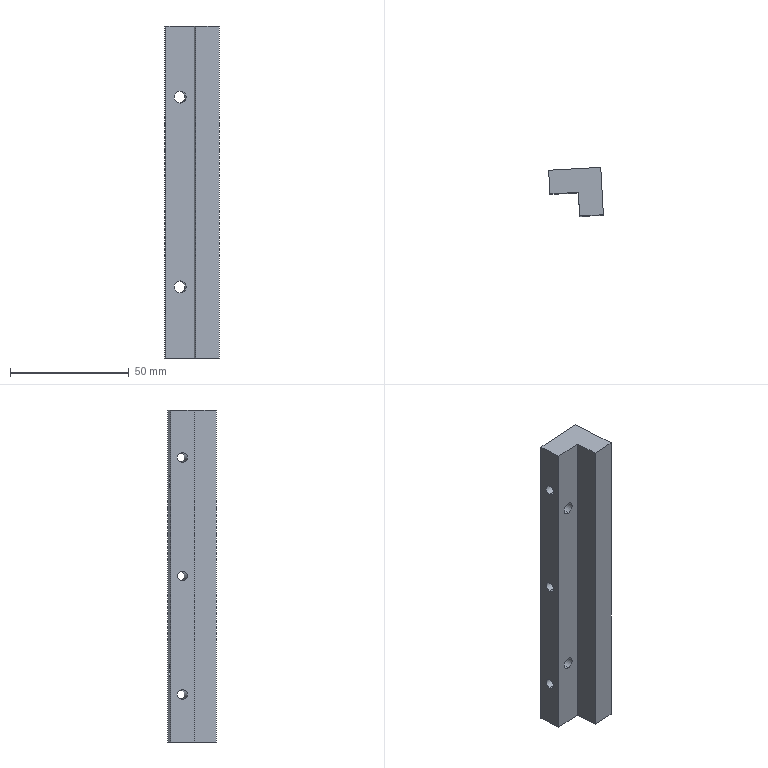Component | SolidWorks | BearingPressPartH-1 | 1 solid | 18 faces | box 23.06 x 20.52 x 140 mm | volume 43493 mm3 | cylinder 10 | plane 8 | commonest cylinder face diameters 4.2 x6 5 x4
build123d program:
from build123d import *

# Parameters (mm, degrees)
BOSS_EXTRUDE1_DEPTH   = 140
M5_TAPPED_HOLE1_D     = 4.2
M6_TAPPED_HOLE1_D     = 5
M6_TAPPED_HOLE1_DEPTH = 36.5
M6_TAPPED_HOLE1_TIP   = 1.502


with BuildPart() as part:
    # Sketch1 → Boss-Extrude1 (new body)
    with BuildSketch(Plane.XY):
        Polygon((0, 0), (10, 0), (10, 20), (-12, 20), (-12, 10), (0, 10), align=None)
    extrude(amount=BOSS_EXTRUDE1_DEPTH)

    # M5 Tapped Hole1 (through all)
    with Locations(Plane(origin=(10, 0, 0), x_dir=(0, 0, -1), z_dir=(1, 0, 0))):
        with Locations((-120, 15), (-70, 15), (-20, 15)):
            Hole(M5_TAPPED_HOLE1_D / 2)

    # M6 Tapped Hole1
    with Locations(Plane(origin=(0, 20, 0), x_dir=(1, 0, 0), z_dir=(0, 1, 0))):
        with Locations((-6, -110), (-6, -30)):
            Hole(M6_TAPPED_HOLE1_D / 2, depth=M6_TAPPED_HOLE1_DEPTH)
            with Locations((0, 0, -(M6_TAPPED_HOLE1_DEPTH + M6_TAPPED_HOLE1_TIP / 2))):  # 118° drill point
                Cone(0, M6_TAPPED_HOLE1_D / 2, M6_TAPPED_HOLE1_TIP, mode=Mode.SUBTRACT)


solid = part.part

# Placed as in the assembly
solid = solid.moved(Location((403.598, 155.593, -283.818), (0, 0, 3.137)))
STEP:
#1=COLOUR_RGB('',0.7922,0.8196,0.9333);
#2=FILL_AREA_STYLE_COLOUR('',#1);
#3=FILL_AREA_STYLE('',(#2));
#4=SURFACE_STYLE_FILL_AREA(#3);
#5=SURFACE_SIDE_STYLE('',(#4));
#6=SURFACE_STYLE_USAGE(.BOTH.,#5);
#7=PRESENTATION_STYLE_ASSIGNMENT((#6));
#8=CARTESIAN_POINT('',(15.632,6.506,-6.942));
#9=VERTEX_POINT('',#8);
#10=CARTESIAN_POINT('',(15.632,6.506,-6.745));
#11=VERTEX_POINT('',#10);
#12=CARTESIAN_POINT('',(15.632,6.506,-6.843));
#13=DIRECTION('',(-0.05472,0.9985,-0.));
#14=DIRECTION('',(0.,0.,1.));
#15=AXIS2_PLACEMENT_3D('',#12,#13,#14);
#16=CIRCLE('',#15,0.09843);
#17=EDGE_CURVE('',#9,#11,#16,.T.);
#18=ORIENTED_EDGE('',*,*,#17,.F.);
#19=CARTESIAN_POINT('',(15.611,6.899,-6.942));
#20=VERTEX_POINT('',#19);
#21=CARTESIAN_POINT('',(15.611,6.899,-6.942));
#22=DIRECTION('',(-0.05472,0.9985,-0.));
#23=VECTOR('',#22,39.37);
#24=LINE('',#21,#23);
#25=EDGE_CURVE('',#9,#20,#24,.T.);
#26=ORIENTED_EDGE('',*,*,#25,.T.);
#27=CARTESIAN_POINT('',(15.611,6.899,-6.745));
#28=VERTEX_POINT('',#27);
#29=CARTESIAN_POINT('',(15.611,6.899,-6.843));
#30=DIRECTION('',(-0.05472,0.9985,-0.));
#31=DIRECTION('',(0.,0.,1.));
#32=AXIS2_PLACEMENT_3D('',#29,#30,#31);
#33=CIRCLE('',#32,0.09843);
#34=EDGE_CURVE('',#20,#28,#33,.T.);
#35=ORIENTED_EDGE('',*,*,#34,.T.);
#36=CARTESIAN_POINT('',(15.611,6.899,-6.745));
#37=DIRECTION('',(-0.05472,0.9985,-0.));
#38=VECTOR('',#37,39.37);
#39=LINE('',#36,#38);
#40=EDGE_CURVE('',#11,#28,#39,.T.);
#41=ORIENTED_EDGE('',*,*,#40,.F.);
#42=EDGE_LOOP('',(#18,#26,#35,#41));
#43=FACE_OUTER_BOUND('',#42,.T.);
#44=CARTESIAN_POINT('',(15.611,6.899,-6.843));
#45=DIRECTION('',(-0.05472,0.9985,-0.));
#46=DIRECTION('',(0.,0.,1.));
#47=AXIS2_PLACEMENT_3D('',#44,#45,#46);
#48=CYLINDRICAL_SURFACE('',#47,0.09843);
#49=ADVANCED_FACE('',(#43),#48,.F.);
#50=CARTESIAN_POINT('',(15.632,6.506,-10.091));
#51=VERTEX_POINT('',#50);
#52=CARTESIAN_POINT('',(15.632,6.506,-9.894));
#53=VERTEX_POINT('',#52);
#54=CARTESIAN_POINT('',(15.632,6.506,-9.993));
#55=DIRECTION('',(-0.05472,0.9985,-0.));
#56=DIRECTION('',(0.,0.,1.));
#57=AXIS2_PLACEMENT_3D('',#54,#55,#56);
#58=CIRCLE('',#57,0.09843);
#59=EDGE_CURVE('',#51,#53,#58,.T.);
#60=ORIENTED_EDGE('',*,*,#59,.F.);
#61=CARTESIAN_POINT('',(15.611,6.899,-10.091));
#62=VERTEX_POINT('',#61);
#63=CARTESIAN_POINT('',(15.611,6.899,-10.091));
#64=DIRECTION('',(-0.05472,0.9985,-0.));
#65=VECTOR('',#64,39.37);
#66=LINE('',#63,#65);
#67=EDGE_CURVE('',#51,#62,#66,.T.);
#68=ORIENTED_EDGE('',*,*,#67,.T.);
#69=CARTESIAN_POINT('',(15.611,6.899,-9.894));
#70=VERTEX_POINT('',#69);
#71=CARTESIAN_POINT('',(15.611,6.899,-9.993));
#72=DIRECTION('',(-0.05472,0.9985,-0.));
#73=DIRECTION('',(0.,0.,1.));
#74=AXIS2_PLACEMENT_3D('',#71,#72,#73);
#75=CIRCLE('',#74,0.09843);
#76=EDGE_CURVE('',#62,#70,#75,.T.);
#77=ORIENTED_EDGE('',*,*,#76,.T.);
#78=CARTESIAN_POINT('',(15.611,6.899,-9.894));
#79=DIRECTION('',(-0.05472,0.9985,-0.));
#80=VECTOR('',#79,39.37);
#81=LINE('',#78,#80);
#82=EDGE_CURVE('',#53,#70,#81,.T.);
#83=ORIENTED_EDGE('',*,*,#82,.F.);
#84=EDGE_LOOP('',(#60,#68,#77,#83));
#85=FACE_OUTER_BOUND('',#84,.T.);
#86=CARTESIAN_POINT('',(15.611,6.899,-9.993));
#87=DIRECTION('',(-0.05472,0.9985,-0.));
#88=DIRECTION('',(0.,0.,1.));
#89=AXIS2_PLACEMENT_3D('',#86,#87,#88);
#90=CYLINDRICAL_SURFACE('',#89,0.09843);
#91=ADVANCED_FACE('',(#85),#90,.F.);
#92=CARTESIAN_POINT('',(15.386,6.69,-6.367));
#93=VERTEX_POINT('',#92);
#94=CARTESIAN_POINT('',(15.386,6.69,-6.532));
#95=VERTEX_POINT('',#94);
#96=CARTESIAN_POINT('',(15.386,6.69,-6.45));
#97=DIRECTION('',(0.9985,0.05472,-0.));
#98=DIRECTION('',(-0.05472,0.9985,0.));
#99=AXIS2_PLACEMENT_3D('',#96,#97,#98);
#100=CIRCLE('',#99,0.08268);
#101=EDGE_CURVE('',#93,#95,#100,.T.);
#102=ORIENTED_EDGE('',*,*,#101,.F.);
#103=CARTESIAN_POINT('',(16.251,6.737,-6.367));
#104=VERTEX_POINT('',#103);
#105=CARTESIAN_POINT('',(16.251,6.737,-6.367));
#106=DIRECTION('',(0.9985,0.05472,-0.));
#107=VECTOR('',#106,39.37);
#108=LINE('',#105,#107);
#109=EDGE_CURVE('',#93,#104,#108,.T.);
#110=ORIENTED_EDGE('',*,*,#109,.T.);
#111=CARTESIAN_POINT('',(16.251,6.737,-6.532));
#112=VERTEX_POINT('',#111);
#113=CARTESIAN_POINT('',(16.251,6.737,-6.45));
#114=DIRECTION('',(0.9985,0.05472,-0.));
#115=DIRECTION('',(0.,0.,-1.));
#116=AXIS2_PLACEMENT_3D('',#113,#114,#115);
#117=CIRCLE('',#116,0.08268);
#118=EDGE_CURVE('',#104,#112,#117,.T.);
#119=ORIENTED_EDGE('',*,*,#118,.T.);
#120=CARTESIAN_POINT('',(16.251,6.737,-6.532));
#121=DIRECTION('',(0.9985,0.05472,-0.));
#122=VECTOR('',#121,39.37);
#123=LINE('',#120,#122);
#124=EDGE_CURVE('',#95,#112,#123,.T.);
#125=ORIENTED_EDGE('',*,*,#124,.F.);
#126=EDGE_LOOP('',(#102,#110,#119,#125));
#127=FACE_OUTER_BOUND('',#126,.T.);
#128=CARTESIAN_POINT('',(16.251,6.737,-6.45));
#129=DIRECTION('',(0.9985,0.05472,-0.));
#130=DIRECTION('',(0.,0.,-1.));
#131=AXIS2_PLACEMENT_3D('',#128,#129,#130);
#132=CYLINDRICAL_SURFACE('',#131,0.08268);
#133=ADVANCED_FACE('',(#127),#132,.F.);
#134=CARTESIAN_POINT('',(15.386,6.69,-8.335));
#135=VERTEX_POINT('',#134);
#136=CARTESIAN_POINT('',(15.386,6.69,-8.501));
#137=VERTEX_POINT('',#136);
#138=CARTESIAN_POINT('',(15.386,6.69,-8.418));
#139=DIRECTION('',(0.9985,0.05472,-0.));
#140=DIRECTION('',(-0.05472,0.9985,0.));
#141=AXIS2_PLACEMENT_3D('',#138,#139,#140);
#142=CIRCLE('',#141,0.08268);
#143=EDGE_CURVE('',#135,#137,#142,.T.);
#144=ORIENTED_EDGE('',*,*,#143,.F.);
#145=CARTESIAN_POINT('',(16.251,6.737,-8.335));
#146=VERTEX_POINT('',#145);
#147=CARTESIAN_POINT('',(16.251,6.737,-8.335));
#148=DIRECTION('',(0.9985,0.05472,-0.));
#149=VECTOR('',#148,39.37);
#150=LINE('',#147,#149);
#151=EDGE_CURVE('',#135,#146,#150,.T.);
#152=ORIENTED_EDGE('',*,*,#151,.T.);
#153=CARTESIAN_POINT('',(16.251,6.737,-8.501));
#154=VERTEX_POINT('',#153);
#155=CARTESIAN_POINT('',(16.251,6.737,-8.418));
#156=DIRECTION('',(0.9985,0.05472,-0.));
#157=DIRECTION('',(0.,0.,-1.));
#158=AXIS2_PLACEMENT_3D('',#155,#156,#157);
#159=CIRCLE('',#158,0.08268);
#160=EDGE_CURVE('',#146,#154,#159,.T.);
#161=ORIENTED_EDGE('',*,*,#160,.T.);
#162=CARTESIAN_POINT('',(16.251,6.737,-8.501));
#163=DIRECTION('',(0.9985,0.05472,-0.));
#164=VECTOR('',#163,39.37);
#165=LINE('',#162,#164);
#166=EDGE_CURVE('',#137,#154,#165,.T.);
#167=ORIENTED_EDGE('',*,*,#166,.F.);
#168=EDGE_LOOP('',(#144,#152,#161,#167));
#169=FACE_OUTER_BOUND('',#168,.T.);
#170=CARTESIAN_POINT('',(16.251,6.737,-8.418));
#171=DIRECTION('',(0.9985,0.05472,-0.));
#172=DIRECTION('',(0.,0.,-1.));
#173=AXIS2_PLACEMENT_3D('',#170,#171,#172);
#174=CYLINDRICAL_SURFACE('',#173,0.08268);
#175=ADVANCED_FACE('',(#169),#174,.F.);
#176=CARTESIAN_POINT('',(15.386,6.69,-10.304));
#177=VERTEX_POINT('',#176);
#178=CARTESIAN_POINT('',(15.386,6.69,-10.469));
#179=VERTEX_POINT('',#178);
#180=CARTESIAN_POINT('',(15.386,6.69,-10.387));
#181=DIRECTION('',(0.9985,0.05472,-0.));
#182=DIRECTION('',(-0.05472,0.9985,0.));
#183=AXIS2_PLACEMENT_3D('',#180,#181,#182);
#184=CIRCLE('',#183,0.08268);
#185=EDGE_CURVE('',#177,#179,#184,.T.);
#186=ORIENTED_EDGE('',*,*,#185,.F.);
#187=CARTESIAN_POINT('',(16.251,6.737,-10.304));
#188=VERTEX_POINT('',#187);
#189=CARTESIAN_POINT('',(16.251,6.737,-10.304));
#190=DIRECTION('',(0.9985,0.05472,-0.));
#191=VECTOR('',#190,39.37);
#192=LINE('',#189,#191);
#193=EDGE_CURVE('',#177,#188,#192,.T.);
#194=ORIENTED_EDGE('',*,*,#193,.T.);
#195=CARTESIAN_POINT('',(16.251,6.737,-10.469));
#196=VERTEX_POINT('',#195);
#197=CARTESIAN_POINT('',(16.251,6.737,-10.387));
#198=DIRECTION('',(0.9985,0.05472,-0.));
#199=DIRECTION('',(0.,0.,-1.));
#200=AXIS2_PLACEMENT_3D('',#197,#198,#199);
#201=CIRCLE('',#200,0.08268);
#202=EDGE_CURVE('',#188,#196,#201,.T.);
#203=ORIENTED_EDGE('',*,*,#202,.T.);
#204=CARTESIAN_POINT('',(16.251,6.737,-10.469));
#205=DIRECTION('',(0.9985,0.05472,-0.));
#206=VECTOR('',#205,39.37);
#207=LINE('',#204,#206);
#208=EDGE_CURVE('',#179,#196,#207,.T.);
#209=ORIENTED_EDGE('',*,*,#208,.F.);
#210=EDGE_LOOP('',(#186,#194,#203,#209));
#211=FACE_OUTER_BOUND('',#210,.T.);
#212=CARTESIAN_POINT('',(16.251,6.737,-10.387));
#213=DIRECTION('',(0.9985,0.05472,-0.));
#214=DIRECTION('',(0.,0.,-1.));
#215=AXIS2_PLACEMENT_3D('',#212,#213,#214);
#216=CYLINDRICAL_SURFACE('',#215,0.08268);
#217=ADVANCED_FACE('',(#211),#216,.F.);
#218=CARTESIAN_POINT('',(16.251,6.737,-10.387));
#219=DIRECTION('',(0.9985,0.05472,-0.));
#220=DIRECTION('',(0.,0.,-1.));
#221=AXIS2_PLACEMENT_3D('',#218,#219,#220);
#222=CIRCLE('',#221,0.08268);
#223=EDGE_CURVE('',#196,#188,#222,.T.);
#224=ORIENTED_EDGE('',*,*,#223,.F.);
#225=ORIENTED_EDGE('',*,*,#202,.F.);
#226=EDGE_LOOP('',(#224,#225));
#227=FACE_BOUND('',#226,.T.);
#228=CARTESIAN_POINT('',(16.283,6.147,-11.174));
#229=VERTEX_POINT('',#228);
#230=CARTESIAN_POINT('',(16.24,6.933,-11.174));
#231=VERTEX_POINT('',#230);
#232=CARTESIAN_POINT('',(16.283,6.147,-11.174));
#233=DIRECTION('',(-0.05472,0.9985,-0.));
#234=VECTOR('',#233,39.37);
#235=LINE('',#232,#234);
#236=EDGE_CURVE('',#229,#231,#235,.T.);
#237=ORIENTED_EDGE('',*,*,#236,.T.);
#238=CARTESIAN_POINT('',(16.24,6.933,-5.662));
#239=VERTEX_POINT('',#238);
#240=CARTESIAN_POINT('',(16.24,6.933,-5.662));
#241=DIRECTION('',(-0.,-0.,-1.));
#242=VECTOR('',#241,39.37);
#243=LINE('',#240,#242);
#244=EDGE_CURVE('',#239,#231,#243,.T.);
#245=ORIENTED_EDGE('',*,*,#244,.F.);
#246=CARTESIAN_POINT('',(16.283,6.147,-5.662));
#247=VERTEX_POINT('',#246);
#248=CARTESIAN_POINT('',(16.283,6.147,-5.662));
#249=DIRECTION('',(-0.05472,0.9985,-0.));
#250=VECTOR('',#249,39.37);
#251=LINE('',#248,#250);
#252=EDGE_CURVE('',#247,#239,#251,.T.);
#253=ORIENTED_EDGE('',*,*,#252,.F.);
#254=CARTESIAN_POINT('',(16.283,6.147,-5.662));
#255=DIRECTION('',(-0.,-0.,-1.));
#256=VECTOR('',#255,39.37);
#257=LINE('',#254,#256);
#258=EDGE_CURVE('',#247,#229,#257,.T.);
#259=ORIENTED_EDGE('',*,*,#258,.T.);
#260=EDGE_LOOP('',(#237,#245,#253,#259));
#261=FACE_OUTER_BOUND('',#260,.T.);
#262=CARTESIAN_POINT('',(16.251,6.737,-8.418));
#263=DIRECTION('',(0.9985,0.05472,-0.));
#264=DIRECTION('',(0.,0.,-1.));
#265=AXIS2_PLACEMENT_3D('',#262,#263,#264);
#266=CIRCLE('',#265,0.08268);
#267=EDGE_CURVE('',#154,#146,#266,.T.);
#268=ORIENTED_EDGE('',*,*,#267,.F.);
#269=ORIENTED_EDGE('',*,*,#160,.F.);
#270=EDGE_LOOP('',(#268,#269));
#271=FACE_BOUND('',#270,.T.);
#272=CARTESIAN_POINT('',(16.251,6.737,-6.45));
#273=DIRECTION('',(0.9985,0.05472,-0.));
#274=DIRECTION('',(0.,0.,-1.));
#275=AXIS2_PLACEMENT_3D('',#272,#273,#274);
#276=CIRCLE('',#275,0.08268);
#277=EDGE_CURVE('',#112,#104,#276,.T.);
#278=ORIENTED_EDGE('',*,*,#277,.F.);
#279=ORIENTED_EDGE('',*,*,#118,.F.);
#280=EDGE_LOOP('',(#278,#279));
#281=FACE_BOUND('',#280,.T.);
#282=CARTESIAN_POINT('',(16.283,6.147,-5.662));
#283=DIRECTION('',(-0.9985,-0.05472,0.));
#284=DIRECTION('',(0.,0.,1.));
#285=AXIS2_PLACEMENT_3D('',#282,#283,#284);
#286=PLANE('',#285);
#287=ADVANCED_FACE('',(#227,#261,#271,#281),#286,.F.);
#288=CARTESIAN_POINT('',(15.868,6.519,-11.174));
#289=VERTEX_POINT('',#288);
#290=CARTESIAN_POINT('',(15.89,6.126,-11.174));
#291=VERTEX_POINT('',#290);
#292=CARTESIAN_POINT('',(15.868,6.519,-11.174));
#293=DIRECTION('',(0.05472,-0.9985,0.));
#294=VECTOR('',#293,39.37);
#295=LINE('',#292,#294);
#296=EDGE_CURVE('',#289,#291,#295,.T.);
#297=ORIENTED_EDGE('',*,*,#296,.T.);
#298=CARTESIAN_POINT('',(15.89,6.126,-5.662));
#299=VERTEX_POINT('',#298);
#300=CARTESIAN_POINT('',(15.89,6.126,-5.662));
#301=DIRECTION('',(-0.,-0.,-1.));
#302=VECTOR('',#301,39.37);
#303=LINE('',#300,#302);
#304=EDGE_CURVE('',#299,#291,#303,.T.);
#305=ORIENTED_EDGE('',*,*,#304,.F.);
#306=CARTESIAN_POINT('',(15.868,6.519,-5.662));
#307=VERTEX_POINT('',#306);
#308=CARTESIAN_POINT('',(15.868,6.519,-5.662));
#309=DIRECTION('',(0.05472,-0.9985,0.));
#310=VECTOR('',#309,39.37);
#311=LINE('',#308,#310);
#312=EDGE_CURVE('',#307,#299,#311,.T.);
#313=ORIENTED_EDGE('',*,*,#312,.F.);
#314=CARTESIAN_POINT('',(15.868,6.519,-5.662));
#315=DIRECTION('',(-0.,-0.,-1.));
#316=VECTOR('',#315,39.37);
#317=LINE('',#314,#316);
#318=EDGE_CURVE('',#307,#289,#317,.T.);
#319=ORIENTED_EDGE('',*,*,#318,.T.);
#320=EDGE_LOOP('',(#297,#305,#313,#319));
#321=FACE_OUTER_BOUND('',#320,.T.);
#322=CARTESIAN_POINT('',(15.868,6.519,-5.662));
#323=DIRECTION('',(0.9985,0.05472,-0.));
#324=DIRECTION('',(-0.05472,0.9985,-0.));
#325=AXIS2_PLACEMENT_3D('',#322,#323,#324);
#326=PLANE('',#325);
#327=ADVANCED_FACE('',(#321),#326,.F.);
#328=CARTESIAN_POINT('',(15.89,6.126,-11.174));
#329=DIRECTION('',(0.9985,0.05472,-0.));
#330=VECTOR('',#329,39.37);
#331=LINE('',#328,#330);
#332=EDGE_CURVE('',#291,#229,#331,.T.);
#333=ORIENTED_EDGE('',*,*,#332,.T.);
#334=ORIENTED_EDGE('',*,*,#258,.F.);
#335=CARTESIAN_POINT('',(15.89,6.126,-5.662));
#336=DIRECTION('',(0.9985,0.05472,-0.));
#337=VECTOR('',#336,39.37);
#338=LINE('',#335,#337);
#339=EDGE_CURVE('',#299,#247,#338,.T.);
#340=ORIENTED_EDGE('',*,*,#339,.F.);
#341=ORIENTED_EDGE('',*,*,#304,.T.);
#342=EDGE_LOOP('',(#333,#334,#340,#341));
#343=FACE_OUTER_BOUND('',#342,.T.);
#344=CARTESIAN_POINT('',(15.89,6.126,-5.662));
#345=DIRECTION('',(-0.05472,0.9985,-0.));
#346=DIRECTION('',(0.,0.,1.));
#347=AXIS2_PLACEMENT_3D('',#344,#345,#346);
#348=PLANE('',#347);
#349=ADVANCED_FACE('',(#343),#348,.F.);
#350=CARTESIAN_POINT('',(15.611,6.899,-6.843));
#351=DIRECTION('',(-0.05472,0.9985,-0.));
#352=DIRECTION('',(0.,0.,1.));
#353=AXIS2_PLACEMENT_3D('',#350,#351,#352);
#354=CIRCLE('',#353,0.09843);
#355=EDGE_CURVE('',#28,#20,#354,.T.);
#356=ORIENTED_EDGE('',*,*,#355,.F.);
#357=ORIENTED_EDGE('',*,*,#34,.F.);
#358=EDGE_LOOP('',(#356,#357));
#359=FACE_BOUND('',#358,.T.);
#360=CARTESIAN_POINT('',(15.611,6.899,-9.993));
#361=DIRECTION('',(-0.05472,0.9985,-0.));
#362=DIRECTION('',(0.,0.,1.));
#363=AXIS2_PLACEMENT_3D('',#360,#361,#362);
#364=CIRCLE('',#363,0.09843);
#365=EDGE_CURVE('',#70,#62,#364,.T.);
#366=ORIENTED_EDGE('',*,*,#365,.F.);
#367=ORIENTED_EDGE('',*,*,#76,.F.);
#368=EDGE_LOOP('',(#366,#367));
#369=FACE_BOUND('',#368,.T.);
#370=CARTESIAN_POINT('',(15.375,6.886,-11.174));
#371=VERTEX_POINT('',#370);
#372=CARTESIAN_POINT('',(16.24,6.933,-11.174));
#373=DIRECTION('',(-0.9985,-0.05472,0.));
#374=VECTOR('',#373,39.37);
#375=LINE('',#372,#374);
#376=EDGE_CURVE('',#231,#371,#375,.T.);
#377=ORIENTED_EDGE('',*,*,#376,.T.);
#378=CARTESIAN_POINT('',(15.375,6.886,-5.662));
#379=VERTEX_POINT('',#378);
#380=CARTESIAN_POINT('',(15.375,6.886,-5.662));
#381=DIRECTION('',(-0.,-0.,-1.));
#382=VECTOR('',#381,39.37);
#383=LINE('',#380,#382);
#384=EDGE_CURVE('',#379,#371,#383,.T.);
#385=ORIENTED_EDGE('',*,*,#384,.F.);
#386=CARTESIAN_POINT('',(16.24,6.933,-5.662));
#387=DIRECTION('',(-0.9985,-0.05472,0.));
#388=VECTOR('',#387,39.37);
#389=LINE('',#386,#388);
#390=EDGE_CURVE('',#239,#379,#389,.T.);
#391=ORIENTED_EDGE('',*,*,#390,.F.);
#392=ORIENTED_EDGE('',*,*,#244,.T.);
#393=EDGE_LOOP('',(#377,#385,#391,#392));
#394=FACE_OUTER_BOUND('',#393,.T.);
#395=CARTESIAN_POINT('',(16.24,6.933,-5.662));
#396=DIRECTION('',(0.05472,-0.9985,0.));
#397=DIRECTION('',(0.9985,0.05472,-0.));
#398=AXIS2_PLACEMENT_3D('',#395,#396,#397);
#399=PLANE('',#398);
#400=ADVANCED_FACE('',(#359,#369,#394),#399,.F.);
#401=CARTESIAN_POINT('',(15.386,6.69,-6.45));
#402=DIRECTION('',(0.9985,0.05472,-0.));
#403=DIRECTION('',(-0.05472,0.9985,0.));
#404=AXIS2_PLACEMENT_3D('',#401,#402,#403);
#405=CIRCLE('',#404,0.08268);
#406=EDGE_CURVE('',#95,#93,#405,.T.);
#407=ORIENTED_EDGE('',*,*,#406,.T.);
#408=ORIENTED_EDGE('',*,*,#101,.T.);
#409=EDGE_LOOP('',(#407,#408));
#410=FACE_BOUND('',#409,.T.);
#411=CARTESIAN_POINT('',(15.386,6.69,-8.418));
#412=DIRECTION('',(0.9985,0.05472,-0.));
#413=DIRECTION('',(-0.05472,0.9985,0.));
#414=AXIS2_PLACEMENT_3D('',#411,#412,#413);
#415=CIRCLE('',#414,0.08268);
#416=EDGE_CURVE('',#137,#135,#415,.T.);
#417=ORIENTED_EDGE('',*,*,#416,.T.);
#418=ORIENTED_EDGE('',*,*,#143,.T.);
#419=EDGE_LOOP('',(#417,#418));
#420=FACE_BOUND('',#419,.T.);
#421=CARTESIAN_POINT('',(15.386,6.69,-10.387));
#422=DIRECTION('',(0.9985,0.05472,-0.));
#423=DIRECTION('',(-0.05472,0.9985,0.));
#424=AXIS2_PLACEMENT_3D('',#421,#422,#423);
#425=CIRCLE('',#424,0.08268);
#426=EDGE_CURVE('',#179,#177,#425,.T.);
#427=ORIENTED_EDGE('',*,*,#426,.T.);
#428=ORIENTED_EDGE('',*,*,#185,.T.);
#429=EDGE_LOOP('',(#427,#428));
#430=FACE_BOUND('',#429,.T.);
#431=CARTESIAN_POINT('',(15.396,6.493,-11.174));
#432=VERTEX_POINT('',#431);
#433=CARTESIAN_POINT('',(15.396,6.493,-11.174));
#434=DIRECTION('',(0.05472,-0.9985,0.));
#435=VECTOR('',#434,39.37);
#436=LINE('',#433,#435);
#437=EDGE_CURVE('',#371,#432,#436,.T.);
#438=ORIENTED_EDGE('',*,*,#437,.T.);
#439=CARTESIAN_POINT('',(15.396,6.493,-5.662));
#440=VERTEX_POINT('',#439);
#441=CARTESIAN_POINT('',(15.396,6.493,-5.662));
#442=DIRECTION('',(-0.,-0.,-1.));
#443=VECTOR('',#442,39.37);
#444=LINE('',#441,#443);
#445=EDGE_CURVE('',#440,#432,#444,.T.);
#446=ORIENTED_EDGE('',*,*,#445,.F.);
#447=CARTESIAN_POINT('',(15.396,6.493,-5.662));
#448=DIRECTION('',(0.05472,-0.9985,0.));
#449=VECTOR('',#448,39.37);
#450=LINE('',#447,#449);
#451=EDGE_CURVE('',#379,#440,#450,.T.);
#452=ORIENTED_EDGE('',*,*,#451,.F.);
#453=ORIENTED_EDGE('',*,*,#384,.T.);
#454=EDGE_LOOP('',(#438,#446,#452,#453));
#455=FACE_OUTER_BOUND('',#454,.T.);
#456=CARTESIAN_POINT('',(15.396,6.493,-5.662));
#457=DIRECTION('',(0.9985,0.05472,-0.));
#458=DIRECTION('',(-0.05472,0.9985,-0.));
#459=AXIS2_PLACEMENT_3D('',#456,#457,#458);
#460=PLANE('',#459);
#461=ADVANCED_FACE('',(#410,#420,#430,#455),#460,.F.);
#462=CARTESIAN_POINT('',(15.632,6.506,-6.843));
#463=DIRECTION('',(-0.05472,0.9985,-0.));
#464=DIRECTION('',(0.,0.,1.));
#465=AXIS2_PLACEMENT_3D('',#462,#463,#464);
#466=CIRCLE('',#465,0.09843);
#467=EDGE_CURVE('',#11,#9,#466,.T.);
#468=ORIENTED_EDGE('',*,*,#467,.T.);
#469=ORIENTED_EDGE('',*,*,#17,.T.);
#470=EDGE_LOOP('',(#468,#469));
#471=FACE_BOUND('',#470,.T.);
#472=CARTESIAN_POINT('',(15.632,6.506,-9.993));
#473=DIRECTION('',(-0.05472,0.9985,-0.));
#474=DIRECTION('',(0.,0.,1.));
#475=AXIS2_PLACEMENT_3D('',#472,#473,#474);
#476=CIRCLE('',#475,0.09843);
#477=EDGE_CURVE('',#53,#51,#476,.T.);
#478=ORIENTED_EDGE('',*,*,#477,.T.);
#479=ORIENTED_EDGE('',*,*,#59,.T.);
#480=EDGE_LOOP('',(#478,#479));
#481=FACE_BOUND('',#480,.T.);
#482=CARTESIAN_POINT('',(15.396,6.493,-11.174));
#483=DIRECTION('',(0.9985,0.05472,-0.));
#484=VECTOR('',#483,39.37);
#485=LINE('',#482,#484);
#486=EDGE_CURVE('',#432,#289,#485,.T.);
#487=ORIENTED_EDGE('',*,*,#486,.T.);
#488=ORIENTED_EDGE('',*,*,#318,.F.);
#489=CARTESIAN_POINT('',(15.396,6.493,-5.662));
#490=DIRECTION('',(0.9985,0.05472,-0.));
#491=VECTOR('',#490,39.37);
#492=LINE('',#489,#491);
#493=EDGE_CURVE('',#440,#307,#492,.T.);
#494=ORIENTED_EDGE('',*,*,#493,.F.);
#495=ORIENTED_EDGE('',*,*,#445,.T.);
#496=EDGE_LOOP('',(#487,#488,#494,#495));
#497=FACE_OUTER_BOUND('',#496,.T.);
#498=CARTESIAN_POINT('',(15.396,6.493,-5.662));
#499=DIRECTION('',(-0.05472,0.9985,-0.));
#500=DIRECTION('',(0.,0.,1.));
#501=AXIS2_PLACEMENT_3D('',#498,#499,#500);
#502=PLANE('',#501);
#503=ADVANCED_FACE('',(#471,#481,#497),#502,.F.);
#504=ORIENTED_EDGE('',*,*,#312,.T.);
#505=ORIENTED_EDGE('',*,*,#339,.T.);
#506=ORIENTED_EDGE('',*,*,#252,.T.);
#507=ORIENTED_EDGE('',*,*,#390,.T.);
#508=ORIENTED_EDGE('',*,*,#451,.T.);
#509=ORIENTED_EDGE('',*,*,#493,.T.);
#510=EDGE_LOOP('',(#504,#505,#506,#507,#508,#509));
#511=FACE_OUTER_BOUND('',#510,.T.);
#512=CARTESIAN_POINT('',(15.89,6.126,-5.662));
#513=DIRECTION('',(0.,0.,1.));
#514=DIRECTION('',(0.9985,0.05472,-0.));
#515=AXIS2_PLACEMENT_3D('',#512,#513,#514);
#516=PLANE('',#515);
#517=ADVANCED_FACE('',(#511),#516,.T.);
#518=ORIENTED_EDGE('',*,*,#296,.F.);
#519=ORIENTED_EDGE('',*,*,#486,.F.);
#520=ORIENTED_EDGE('',*,*,#437,.F.);
#521=ORIENTED_EDGE('',*,*,#376,.F.);
#522=ORIENTED_EDGE('',*,*,#236,.F.);
#523=ORIENTED_EDGE('',*,*,#332,.F.);
#524=EDGE_LOOP('',(#518,#519,#520,#521,#522,#523));
#525=FACE_OUTER_BOUND('',#524,.T.);
#526=CARTESIAN_POINT('',(15.89,6.126,-11.174));
#527=DIRECTION('',(0.,0.,1.));
#528=DIRECTION('',(0.9985,0.05472,-0.));
#529=AXIS2_PLACEMENT_3D('',#526,#527,#528);
#530=PLANE('',#529);
#531=ADVANCED_FACE('',(#525),#530,.F.);
#532=ORIENTED_EDGE('',*,*,#193,.F.);
#533=ORIENTED_EDGE('',*,*,#426,.F.);
#534=ORIENTED_EDGE('',*,*,#208,.T.);
#535=ORIENTED_EDGE('',*,*,#223,.T.);
#536=EDGE_LOOP('',(#532,#533,#534,#535));
#537=FACE_OUTER_BOUND('',#536,.T.);
#538=CARTESIAN_POINT('',(16.251,6.737,-10.387));
#539=DIRECTION('',(0.9985,0.05472,-0.));
#540=DIRECTION('',(0.,0.,-1.));
#541=AXIS2_PLACEMENT_3D('',#538,#539,#540);
#542=CYLINDRICAL_SURFACE('',#541,0.08268);
#543=ADVANCED_FACE('',(#537),#542,.F.);
#544=ORIENTED_EDGE('',*,*,#151,.F.);
#545=ORIENTED_EDGE('',*,*,#416,.F.);
#546=ORIENTED_EDGE('',*,*,#166,.T.);
#547=ORIENTED_EDGE('',*,*,#267,.T.);
#548=EDGE_LOOP('',(#544,#545,#546,#547));
#549=FACE_OUTER_BOUND('',#548,.T.);
#550=CARTESIAN_POINT('',(16.251,6.737,-8.418));
#551=DIRECTION('',(0.9985,0.05472,-0.));
#552=DIRECTION('',(0.,0.,-1.));
#553=AXIS2_PLACEMENT_3D('',#550,#551,#552);
#554=CYLINDRICAL_SURFACE('',#553,0.08268);
#555=ADVANCED_FACE('',(#549),#554,.F.);
#556=ORIENTED_EDGE('',*,*,#109,.F.);
#557=ORIENTED_EDGE('',*,*,#406,.F.);
#558=ORIENTED_EDGE('',*,*,#124,.T.);
#559=ORIENTED_EDGE('',*,*,#277,.T.);
#560=EDGE_LOOP('',(#556,#557,#558,#559));
#561=FACE_OUTER_BOUND('',#560,.T.);
#562=CARTESIAN_POINT('',(16.251,6.737,-6.45));
#563=DIRECTION('',(0.9985,0.05472,-0.));
#564=DIRECTION('',(0.,0.,-1.));
#565=AXIS2_PLACEMENT_3D('',#562,#563,#564);
#566=CYLINDRICAL_SURFACE('',#565,0.08268);
#567=ADVANCED_FACE('',(#561),#566,.F.);
#568=ORIENTED_EDGE('',*,*,#67,.F.);
#569=ORIENTED_EDGE('',*,*,#477,.F.);
#570=ORIENTED_EDGE('',*,*,#82,.T.);
#571=ORIENTED_EDGE('',*,*,#365,.T.);
#572=EDGE_LOOP('',(#568,#569,#570,#571));
#573=FACE_OUTER_BOUND('',#572,.T.);
#574=CARTESIAN_POINT('',(15.611,6.899,-9.993));
#575=DIRECTION('',(-0.05472,0.9985,-0.));
#576=DIRECTION('',(0.,0.,1.));
#577=AXIS2_PLACEMENT_3D('',#574,#575,#576);
#578=CYLINDRICAL_SURFACE('',#577,0.09843);
#579=ADVANCED_FACE('',(#573),#578,.F.);
#580=ORIENTED_EDGE('',*,*,#25,.F.);
#581=ORIENTED_EDGE('',*,*,#467,.F.);
#582=ORIENTED_EDGE('',*,*,#40,.T.);
#583=ORIENTED_EDGE('',*,*,#355,.T.);
#584=EDGE_LOOP('',(#580,#581,#582,#583));
#585=FACE_OUTER_BOUND('',#584,.T.);
#586=CARTESIAN_POINT('',(15.611,6.899,-6.843));
#587=DIRECTION('',(-0.05472,0.9985,-0.));
#588=DIRECTION('',(0.,0.,1.));
#589=AXIS2_PLACEMENT_3D('',#586,#587,#588);
#590=CYLINDRICAL_SURFACE('',#589,0.09843);
#591=ADVANCED_FACE('',(#585),#590,.F.);
#592=CLOSED_SHELL('',(#49,#91,#133,#175,#217,#287,#327,#349,#400,#461,#503,#517,#531,#543,#555,#567,#579,#591));
#593=MANIFOLD_SOLID_BREP('',#592);
#594=STYLED_ITEM('',(#7),#593);
#595=PRESENTATION_LAYER_ASSIGNMENT('','',(#594));
#596=CARTESIAN_POINT('',(0.,0.,0.));
#597=DIRECTION('',(0.,0.,1.));
#598=DIRECTION('',(1.,0.,0.));
#599=AXIS2_PLACEMENT_3D('',#596,#597,#598);
#600=(LENGTH_UNIT()NAMED_UNIT(*)SI_UNIT($,.METRE.));
#601=LENGTH_MEASURE_WITH_UNIT(LENGTH_MEASURE(0.0254),#600);
#602=DIMENSIONAL_EXPONENTS(1.,0.,0.,0.,0.,0.,0.);
#603=(CONVERSION_BASED_UNIT('',#601)LENGTH_UNIT()NAMED_UNIT(#602));
#604=UNCERTAINTY_MEASURE_WITH_UNIT(LENGTH_MEASURE(0.00001),#603,'','');
#605=(NAMED_UNIT(*)PLANE_ANGLE_UNIT()SI_UNIT($,.RADIAN.));
#606=(NAMED_UNIT(*)SI_UNIT($,.STERADIAN.)SOLID_ANGLE_UNIT());
#607=(GEOMETRIC_REPRESENTATION_CONTEXT(3)GLOBAL_UNCERTAINTY_ASSIGNED_CONTEXT((#604))GLOBAL_UNIT_ASSIGNED_CONTEXT((#603,#605,#606))REPRESENTATION_CONTEXT('',''));
#608=ADVANCED_BREP_SHAPE_REPRESENTATION('',(#593,#599),#607);
#609=(LENGTH_UNIT()NAMED_UNIT(*)SI_UNIT($,.METRE.));
#610=LENGTH_MEASURE_WITH_UNIT(LENGTH_MEASURE(0.0254),#609);
#611=DIMENSIONAL_EXPONENTS(1.,0.,0.,0.,0.,0.,0.);
#612=(CONVERSION_BASED_UNIT('',#610)LENGTH_UNIT()NAMED_UNIT(#611));
#613=UNCERTAINTY_MEASURE_WITH_UNIT(LENGTH_MEASURE(0.00001),#612,'','');
#614=(NAMED_UNIT(*)PLANE_ANGLE_UNIT()SI_UNIT($,.RADIAN.));
#615=(NAMED_UNIT(*)SI_UNIT($,.STERADIAN.)SOLID_ANGLE_UNIT());
#616=(GEOMETRIC_REPRESENTATION_CONTEXT(3)GLOBAL_UNCERTAINTY_ASSIGNED_CONTEXT((#613))GLOBAL_UNIT_ASSIGNED_CONTEXT((#612,#614,#615))REPRESENTATION_CONTEXT('',''));
#617=MECHANICAL_DESIGN_GEOMETRIC_PRESENTATION_REPRESENTATION('',(#594),#616);